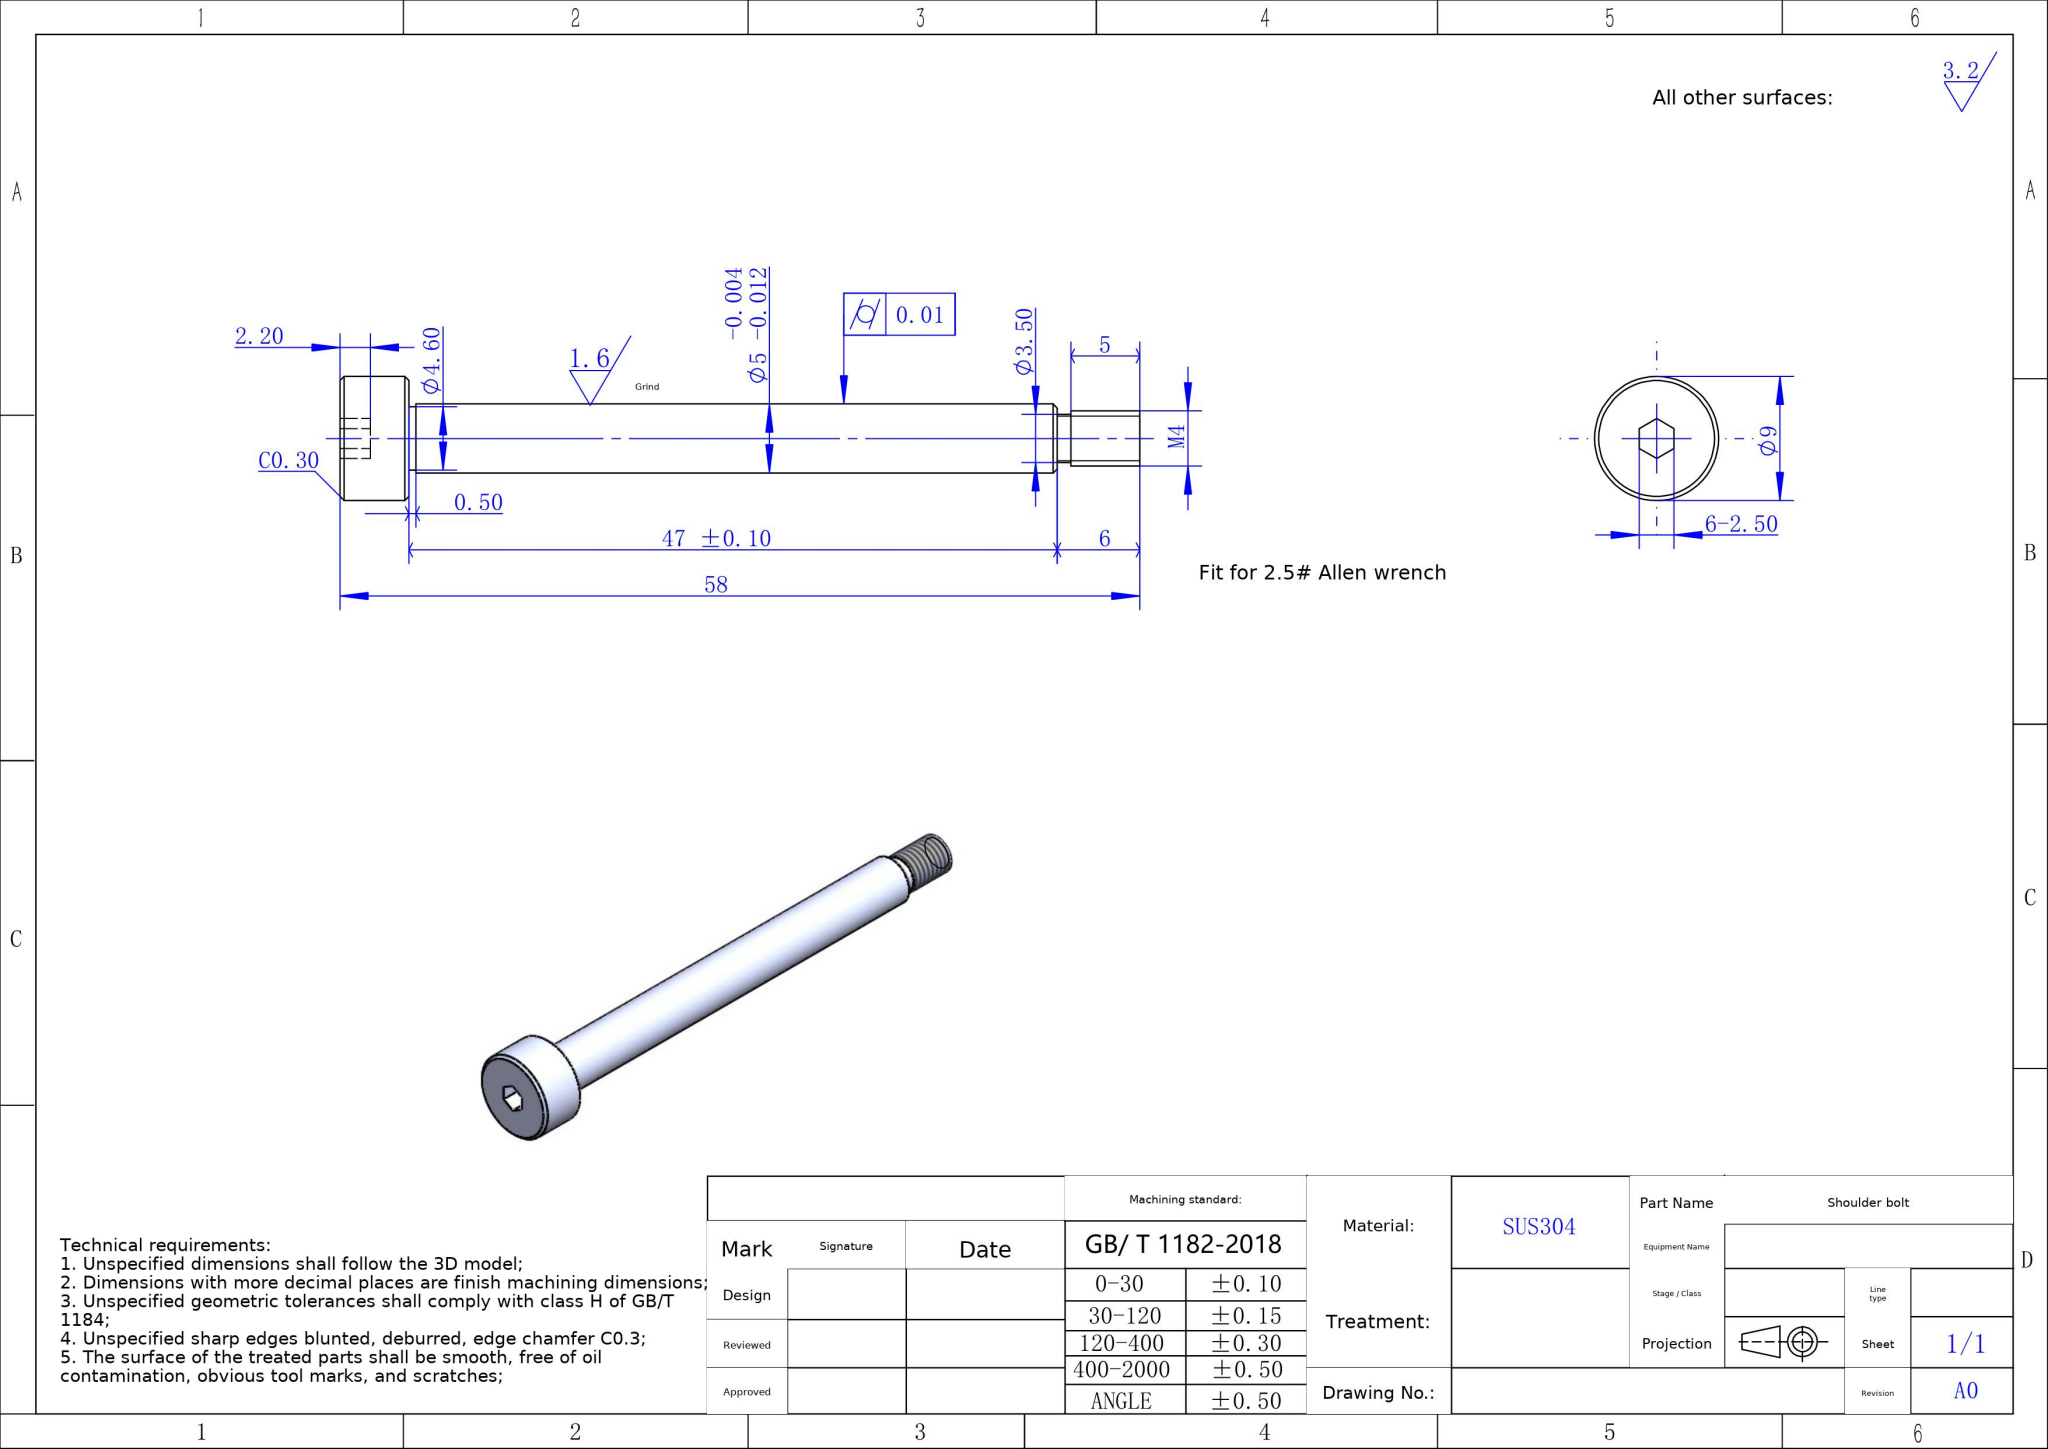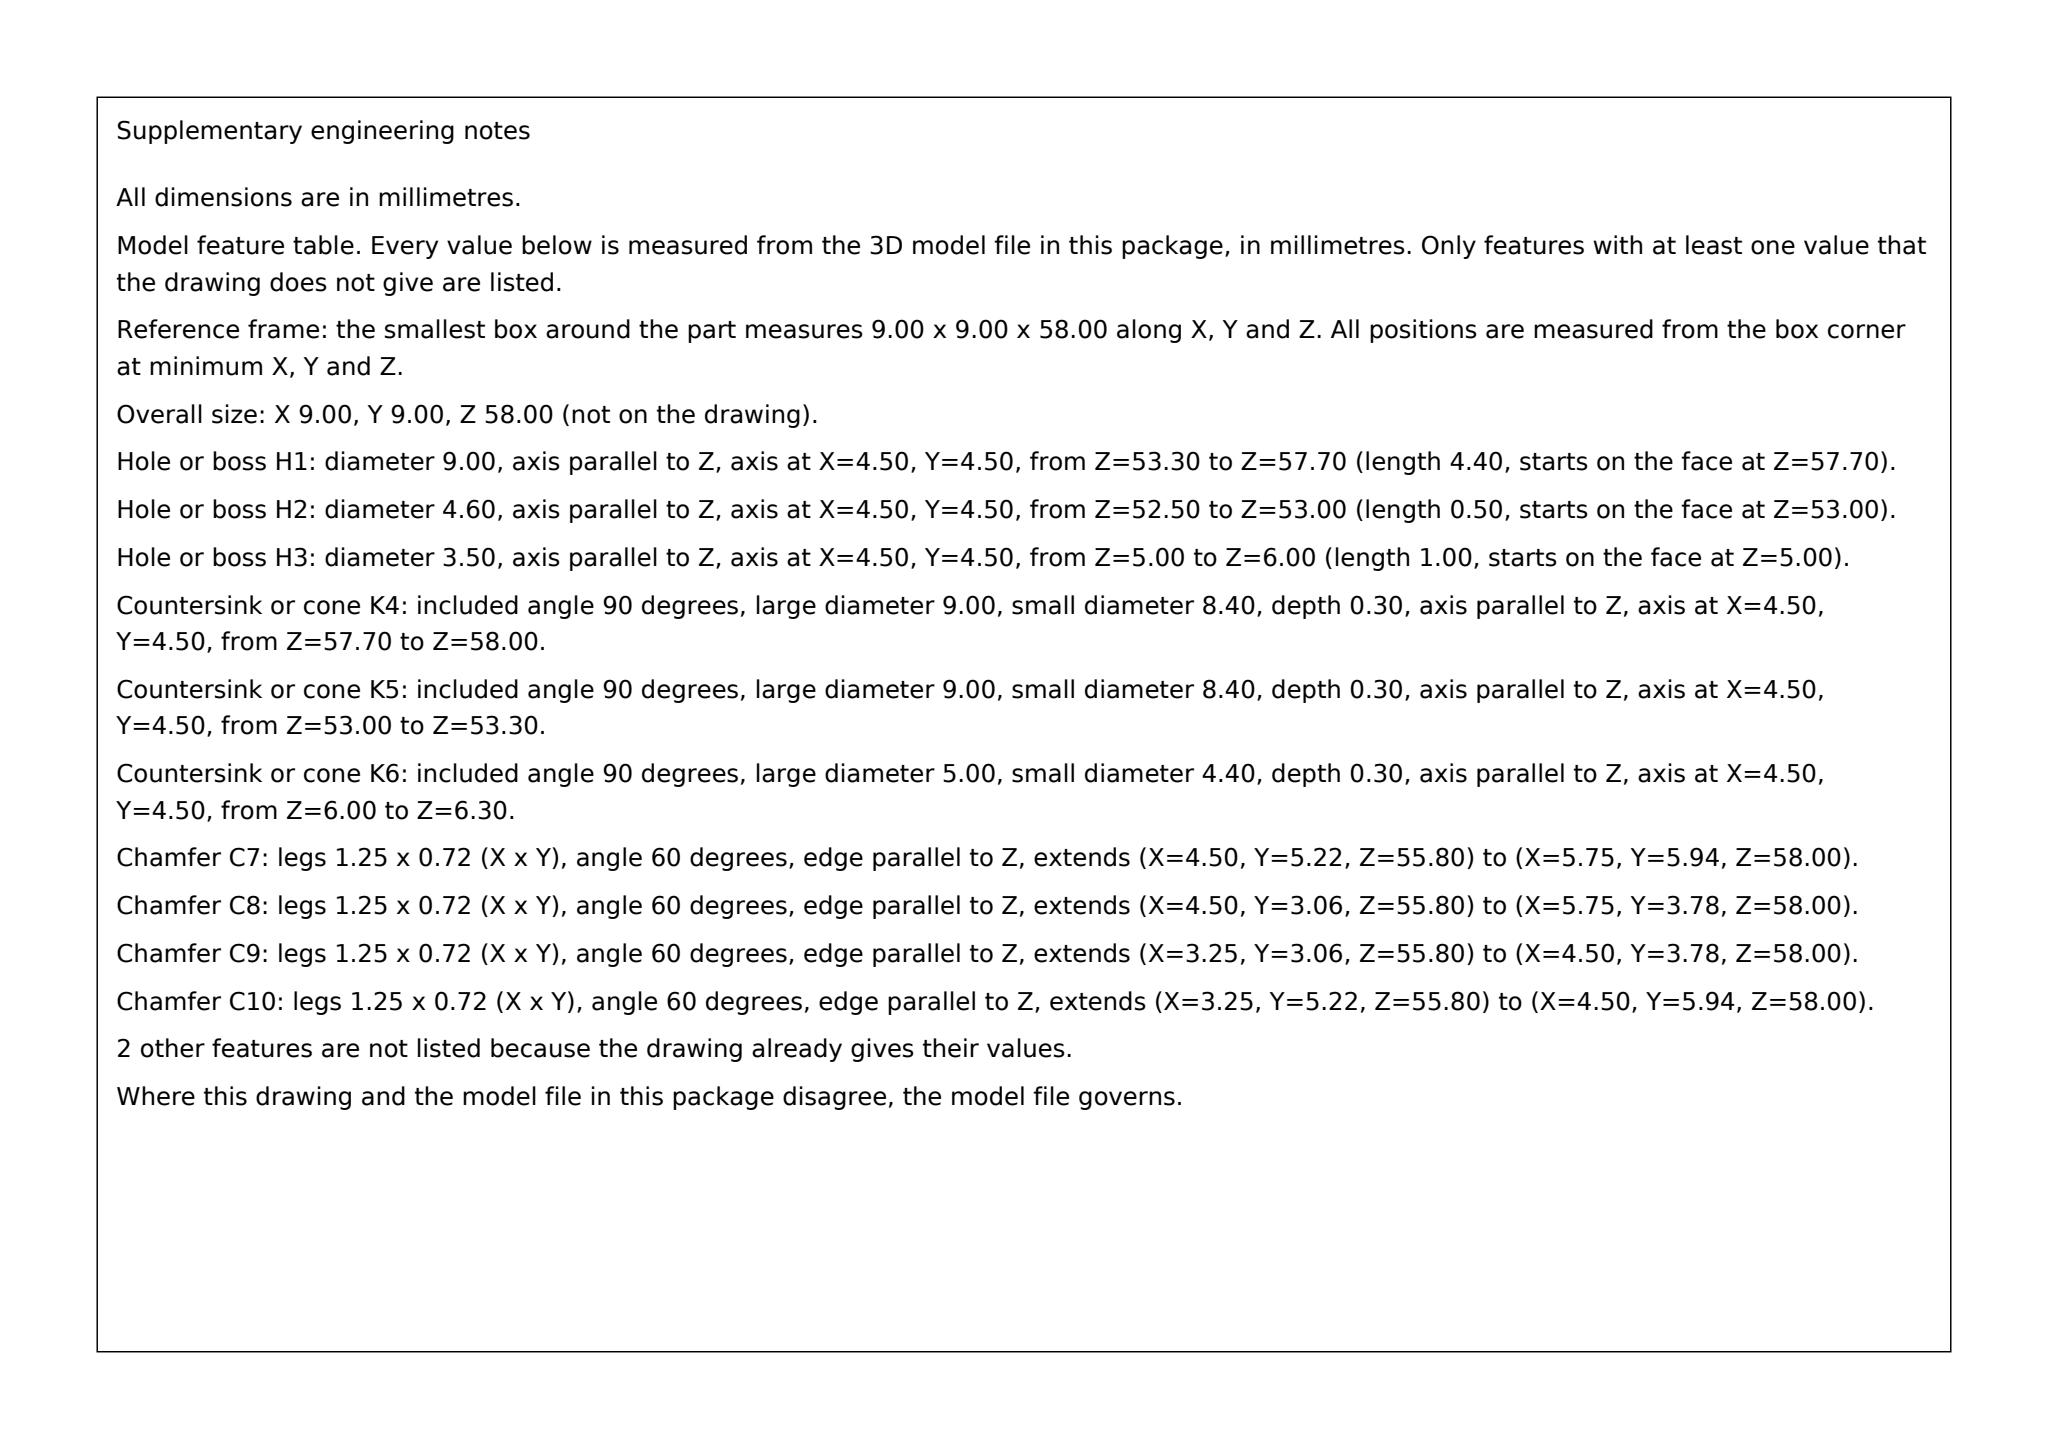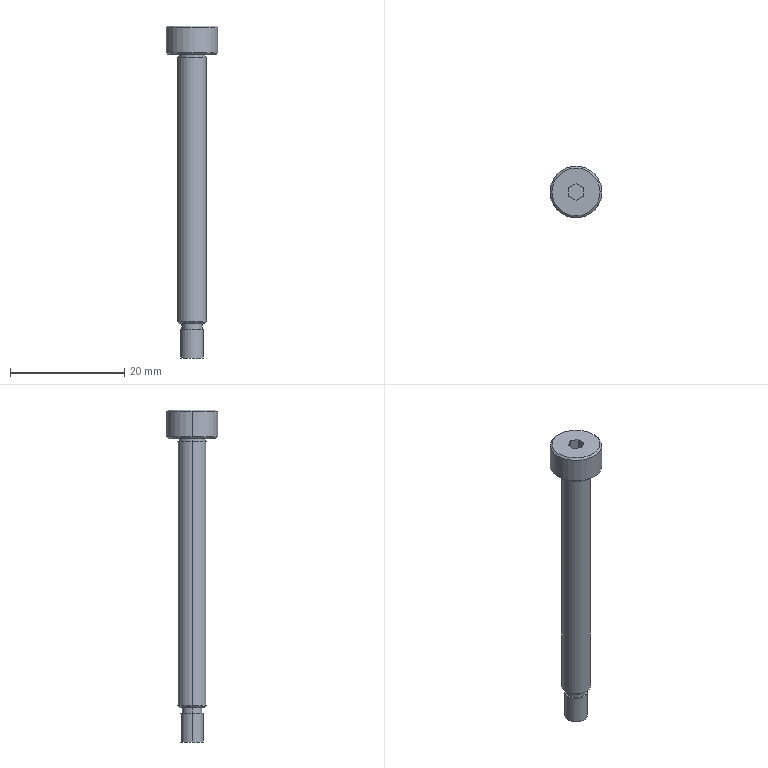Part | SolidWorks | mm | material SUS304 | 1 solid | 29 faces | box 9 x 9 x 58 mm | volume 1297 mm3 | plane 13 | cylinder 10 | cone 6 | commonest cylinder face diameters 4 x2 3.5 x2 5 x2 4.6 x2 9 x2
build123d program:
from build123d import *

# Parameters (mm, degrees)
SKETCH1_R           = 4.5
BOSS_EXTRUDE1_DEPTH = 5
SKETCH2_R           = 2.5
BOSS_EXTRUDE2_DEPTH = 47
SKETCH3_R           = 2
BOSS_EXTRUDE3_DEPTH = 6
SKETCH4_W           = 0.486
SKETCH4_H           = 1
SKETCH4_W_2         = 0.3002
SKETCH4_H_2         = 0.5
CUT_EXTRUDE1_DEPTH  = 2.2
CHAMFER1_SIZE       = 0.3


with BuildPart() as part:
    # Sketch1 → Boss-Extrude1 (new body)
    with BuildSketch(Plane.XY):
        Circle(SKETCH1_R)
    extrude(amount=BOSS_EXTRUDE1_DEPTH)

    # Sketch2 → Boss-Extrude2 (add)
    with BuildSketch(Plane(origin=(0, 0, 0), x_dir=(-1, 0, 0), z_dir=(0, 0, -1))):
        Circle(SKETCH2_R)
    extrude(amount=BOSS_EXTRUDE2_DEPTH)

    # Sketch3 → Boss-Extrude3 (add)
    with BuildSketch(Plane(origin=(0, 0, -47), x_dir=(-1, 0, 0), z_dir=(0, 0, -1))):
        Circle(SKETCH3_R)
    extrude(amount=BOSS_EXTRUDE3_DEPTH)

    # Sketch4 → Cut-Revolve1 (revolve, cut)
    with BuildSketch(Plane(origin=(0, 0, 0), x_dir=(1, 0, 0), z_dir=(0, 1, 0))):
        with Locations((1.993, 47.5)):
            Rectangle(SKETCH4_W, SKETCH4_H)
        with Locations((2.45, 0.25)):
            Rectangle(SKETCH4_W_2, SKETCH4_H_2)
    revolve(axis=Axis((0, 0, -53), (0, 0, -1)), mode=Mode.SUBTRACT)

    # Sketch5 → Cut-Extrude1 (cut)
    with BuildSketch(Plane.XY.offset(5)):
        Polygon((0, 1.443), (-1.25, 0.7217), (-1.25, -0.7217), (0, -1.443), (1.25, -0.7217), (1.25, 0.7217), align=None)
    extrude(amount=-CUT_EXTRUDE1_DEPTH, mode=Mode.SUBTRACT)

    # Chamfer1
    chamfer1_edges = [part.edges().sort_by_distance(p)[0] for p in [
        (-4.5, 0, 0),
        (-4.5, 0, 5),
        (2.5, 0, -47),
    ]]
    chamfer(chamfer1_edges, length=CHAMFER1_SIZE)


solid = part.part
STEP:
#1=CARTESIAN_POINT('',(4.2,0.,5.));
#2=VERTEX_POINT('',#1);
#3=CARTESIAN_POINT('',(-4.2,0.,5.));
#4=VERTEX_POINT('',#3);
#5=CARTESIAN_POINT('',(0.,0.,5.));
#6=DIRECTION('',(0.,0.,1.));
#7=DIRECTION('',(1.,0.,0.));
#8=AXIS2_PLACEMENT_3D('',#5,#6,#7);
#9=CIRCLE('',#8,4.2);
#10=EDGE_CURVE('',#2,#4,#9,.T.);
#11=ORIENTED_EDGE('',*,*,#10,.F.);
#12=CARTESIAN_POINT('',(4.5,0.,4.7));
#13=VERTEX_POINT('',#12);
#14=CARTESIAN_POINT('',(4.2,0.,5.));
#15=DIRECTION('',(0.7071,0.,-0.7071));
#16=VECTOR('',#15,1000.);
#17=LINE('',#14,#16);
#18=EDGE_CURVE('',#2,#13,#17,.T.);
#19=ORIENTED_EDGE('',*,*,#18,.T.);
#20=CARTESIAN_POINT('',(-4.5,0.,4.7));
#21=VERTEX_POINT('',#20);
#22=CARTESIAN_POINT('',(0.,0.,4.7));
#23=DIRECTION('',(0.,0.,-1.));
#24=DIRECTION('',(1.,0.,0.));
#25=AXIS2_PLACEMENT_3D('',#22,#23,#24);
#26=CIRCLE('',#25,4.5);
#27=EDGE_CURVE('',#21,#13,#26,.T.);
#28=ORIENTED_EDGE('',*,*,#27,.F.);
#29=CARTESIAN_POINT('',(-4.2,0.,5.));
#30=DIRECTION('',(-0.7071,0.,-0.7071));
#31=VECTOR('',#30,1000.);
#32=LINE('',#29,#31);
#33=EDGE_CURVE('',#4,#21,#32,.T.);
#34=ORIENTED_EDGE('',*,*,#33,.F.);
#35=EDGE_LOOP('',(#11,#19,#28,#34));
#36=FACE_OUTER_BOUND('',#35,.T.);
#37=CARTESIAN_POINT('',(0.,0.,5.));
#38=DIRECTION('',(0.,0.,-1.));
#39=DIRECTION('',(-1.,0.,0.));
#40=AXIS2_PLACEMENT_3D('',#37,#38,#39);
#41=CONICAL_SURFACE('',#40,4.2,0.7854);
#42=ADVANCED_FACE('',(#36),#41,.T.);
#43=CARTESIAN_POINT('',(-4.2,0.,0.));
#44=VERTEX_POINT('',#43);
#45=CARTESIAN_POINT('',(4.2,0.,0.));
#46=VERTEX_POINT('',#45);
#47=CARTESIAN_POINT('',(0.,0.,0.));
#48=DIRECTION('',(0.,0.,-1.));
#49=DIRECTION('',(1.,0.,0.));
#50=AXIS2_PLACEMENT_3D('',#47,#48,#49);
#51=CIRCLE('',#50,4.2);
#52=EDGE_CURVE('',#44,#46,#51,.T.);
#53=ORIENTED_EDGE('',*,*,#52,.F.);
#54=CARTESIAN_POINT('',(-4.5,0.,0.3));
#55=VERTEX_POINT('',#54);
#56=CARTESIAN_POINT('',(-4.5,0.,0.3));
#57=DIRECTION('',(-0.7071,0.,0.7071));
#58=VECTOR('',#57,1000.);
#59=LINE('',#56,#58);
#60=EDGE_CURVE('',#44,#55,#59,.T.);
#61=ORIENTED_EDGE('',*,*,#60,.T.);
#62=CARTESIAN_POINT('',(4.5,0.,0.3));
#63=VERTEX_POINT('',#62);
#64=CARTESIAN_POINT('',(0.,0.,0.3));
#65=DIRECTION('',(0.,0.,1.));
#66=DIRECTION('',(1.,0.,0.));
#67=AXIS2_PLACEMENT_3D('',#64,#65,#66);
#68=CIRCLE('',#67,4.5);
#69=EDGE_CURVE('',#63,#55,#68,.T.);
#70=ORIENTED_EDGE('',*,*,#69,.F.);
#71=CARTESIAN_POINT('',(4.5,0.,0.3));
#72=DIRECTION('',(0.7071,0.,0.7071));
#73=VECTOR('',#72,1000.);
#74=LINE('',#71,#73);
#75=EDGE_CURVE('',#46,#63,#74,.T.);
#76=ORIENTED_EDGE('',*,*,#75,.F.);
#77=EDGE_LOOP('',(#53,#61,#70,#76));
#78=FACE_OUTER_BOUND('',#77,.T.);
#79=CARTESIAN_POINT('',(0.,0.,0.3));
#80=DIRECTION('',(0.,0.,1.));
#81=DIRECTION('',(1.,0.,0.));
#82=AXIS2_PLACEMENT_3D('',#79,#80,#81);
#83=CONICAL_SURFACE('',#82,4.5,0.7854);
#84=ADVANCED_FACE('',(#78),#83,.T.);
#85=CARTESIAN_POINT('',(-2.2,0.,-47.));
#86=VERTEX_POINT('',#85);
#87=CARTESIAN_POINT('',(2.2,0.,-47.));
#88=VERTEX_POINT('',#87);
#89=CARTESIAN_POINT('',(0.,0.,-47.));
#90=DIRECTION('',(0.,0.,-1.));
#91=DIRECTION('',(-1.,0.,0.));
#92=AXIS2_PLACEMENT_3D('',#89,#90,#91);
#93=CIRCLE('',#92,2.2);
#94=EDGE_CURVE('',#86,#88,#93,.T.);
#95=ORIENTED_EDGE('',*,*,#94,.F.);
#96=CARTESIAN_POINT('',(-2.5,0.,-46.7));
#97=VERTEX_POINT('',#96);
#98=CARTESIAN_POINT('',(-2.2,0.,-47.));
#99=DIRECTION('',(-0.7071,0.,0.7071));
#100=VECTOR('',#99,1000.);
#101=LINE('',#98,#100);
#102=EDGE_CURVE('',#86,#97,#101,.T.);
#103=ORIENTED_EDGE('',*,*,#102,.T.);
#104=CARTESIAN_POINT('',(2.5,0.,-46.7));
#105=VERTEX_POINT('',#104);
#106=CARTESIAN_POINT('',(0.,0.,-46.7));
#107=DIRECTION('',(0.,0.,1.));
#108=DIRECTION('',(-1.,0.,0.));
#109=AXIS2_PLACEMENT_3D('',#106,#107,#108);
#110=CIRCLE('',#109,2.5);
#111=EDGE_CURVE('',#105,#97,#110,.T.);
#112=ORIENTED_EDGE('',*,*,#111,.F.);
#113=CARTESIAN_POINT('',(2.2,0.,-47.));
#114=DIRECTION('',(0.7071,0.,0.7071));
#115=VECTOR('',#114,1000.);
#116=LINE('',#113,#115);
#117=EDGE_CURVE('',#88,#105,#116,.T.);
#118=ORIENTED_EDGE('',*,*,#117,.F.);
#119=EDGE_LOOP('',(#95,#103,#112,#118));
#120=FACE_OUTER_BOUND('',#119,.T.);
#121=CARTESIAN_POINT('',(0.,0.,-47.));
#122=DIRECTION('',(0.,0.,1.));
#123=DIRECTION('',(1.,0.,0.));
#124=AXIS2_PLACEMENT_3D('',#121,#122,#123);
#125=CONICAL_SURFACE('',#124,2.2,0.7854);
#126=ADVANCED_FACE('',(#120),#125,.T.);
#127=CARTESIAN_POINT('',(-2.,0.,-53.));
#128=VERTEX_POINT('',#127);
#129=CARTESIAN_POINT('',(2.,0.,-53.));
#130=VERTEX_POINT('',#129);
#131=CARTESIAN_POINT('',(0.,0.,-53.));
#132=DIRECTION('',(0.,0.,-1.));
#133=DIRECTION('',(-1.,0.,0.));
#134=AXIS2_PLACEMENT_3D('',#131,#132,#133);
#135=CIRCLE('',#134,2.);
#136=EDGE_CURVE('',#128,#130,#135,.T.);
#137=ORIENTED_EDGE('',*,*,#136,.F.);
#138=CARTESIAN_POINT('',(-2.,0.,-48.));
#139=VERTEX_POINT('',#138);
#140=CARTESIAN_POINT('',(-2.,0.,-53.));
#141=DIRECTION('',(0.,0.,1.));
#142=VECTOR('',#141,1000.);
#143=LINE('',#140,#142);
#144=EDGE_CURVE('',#128,#139,#143,.T.);
#145=ORIENTED_EDGE('',*,*,#144,.T.);
#146=CARTESIAN_POINT('',(2.,0.,-48.));
#147=VERTEX_POINT('',#146);
#148=CARTESIAN_POINT('',(0.,0.,-48.));
#149=DIRECTION('',(0.,0.,-1.));
#150=DIRECTION('',(-1.,0.,0.));
#151=AXIS2_PLACEMENT_3D('',#148,#149,#150);
#152=CIRCLE('',#151,2.);
#153=EDGE_CURVE('',#139,#147,#152,.T.);
#154=ORIENTED_EDGE('',*,*,#153,.T.);
#155=CARTESIAN_POINT('',(2.,0.,-53.));
#156=DIRECTION('',(0.,0.,1.));
#157=VECTOR('',#156,1000.);
#158=LINE('',#155,#157);
#159=EDGE_CURVE('',#130,#147,#158,.T.);
#160=ORIENTED_EDGE('',*,*,#159,.F.);
#161=EDGE_LOOP('',(#137,#145,#154,#160));
#162=FACE_OUTER_BOUND('',#161,.T.);
#163=CARTESIAN_POINT('',(0.,0.,-53.));
#164=DIRECTION('',(0.,0.,1.));
#165=DIRECTION('',(1.,0.,0.));
#166=AXIS2_PLACEMENT_3D('',#163,#164,#165);
#167=CYLINDRICAL_SURFACE('',#166,2.);
#168=ADVANCED_FACE('',(#162),#167,.T.);
#169=CARTESIAN_POINT('',(1.75,0.,-48.));
#170=VERTEX_POINT('',#169);
#171=CARTESIAN_POINT('',(-1.75,0.,-48.));
#172=VERTEX_POINT('',#171);
#173=CARTESIAN_POINT('',(0.,0.,-48.));
#174=DIRECTION('',(0.,0.,1.));
#175=DIRECTION('',(1.,0.,0.));
#176=AXIS2_PLACEMENT_3D('',#173,#174,#175);
#177=CIRCLE('',#176,1.75);
#178=EDGE_CURVE('',#170,#172,#177,.T.);
#179=ORIENTED_EDGE('',*,*,#178,.T.);
#180=CARTESIAN_POINT('',(-1.75,0.,-47.));
#181=VERTEX_POINT('',#180);
#182=CARTESIAN_POINT('',(-1.75,0.,-53.));
#183=DIRECTION('',(0.,0.,1.));
#184=VECTOR('',#183,1000.);
#185=LINE('',#182,#184);
#186=EDGE_CURVE('',#172,#181,#185,.T.);
#187=ORIENTED_EDGE('',*,*,#186,.T.);
#188=CARTESIAN_POINT('',(1.75,0.,-47.));
#189=VERTEX_POINT('',#188);
#190=CARTESIAN_POINT('',(0.,0.,-47.));
#191=DIRECTION('',(0.,0.,1.));
#192=DIRECTION('',(1.,0.,0.));
#193=AXIS2_PLACEMENT_3D('',#190,#191,#192);
#194=CIRCLE('',#193,1.75);
#195=EDGE_CURVE('',#189,#181,#194,.T.);
#196=ORIENTED_EDGE('',*,*,#195,.F.);
#197=CARTESIAN_POINT('',(1.75,0.,-53.));
#198=DIRECTION('',(0.,0.,1.));
#199=VECTOR('',#198,1000.);
#200=LINE('',#197,#199);
#201=EDGE_CURVE('',#170,#189,#200,.T.);
#202=ORIENTED_EDGE('',*,*,#201,.F.);
#203=EDGE_LOOP('',(#179,#187,#196,#202));
#204=FACE_OUTER_BOUND('',#203,.T.);
#205=CARTESIAN_POINT('',(0.,0.,-53.));
#206=DIRECTION('',(0.,0.,1.));
#207=DIRECTION('',(1.,0.,0.));
#208=AXIS2_PLACEMENT_3D('',#205,#206,#207);
#209=CYLINDRICAL_SURFACE('',#208,1.75);
#210=ADVANCED_FACE('',(#204),#209,.T.);
#211=ORIENTED_EDGE('',*,*,#111,.T.);
#212=CARTESIAN_POINT('',(-2.5,0.,-0.5));
#213=VERTEX_POINT('',#212);
#214=CARTESIAN_POINT('',(-2.5,0.,-47.));
#215=DIRECTION('',(0.,0.,1.));
#216=VECTOR('',#215,1000.);
#217=LINE('',#214,#216);
#218=EDGE_CURVE('',#97,#213,#217,.T.);
#219=ORIENTED_EDGE('',*,*,#218,.T.);
#220=CARTESIAN_POINT('',(2.5,0.,-0.5));
#221=VERTEX_POINT('',#220);
#222=CARTESIAN_POINT('',(0.,0.,-0.5));
#223=DIRECTION('',(0.,0.,-1.));
#224=DIRECTION('',(-1.,0.,0.));
#225=AXIS2_PLACEMENT_3D('',#222,#223,#224);
#226=CIRCLE('',#225,2.5);
#227=EDGE_CURVE('',#213,#221,#226,.T.);
#228=ORIENTED_EDGE('',*,*,#227,.T.);
#229=CARTESIAN_POINT('',(2.5,0.,-47.));
#230=DIRECTION('',(0.,0.,1.));
#231=VECTOR('',#230,1000.);
#232=LINE('',#229,#231);
#233=EDGE_CURVE('',#105,#221,#232,.T.);
#234=ORIENTED_EDGE('',*,*,#233,.F.);
#235=EDGE_LOOP('',(#211,#219,#228,#234));
#236=FACE_OUTER_BOUND('',#235,.T.);
#237=CARTESIAN_POINT('',(0.,0.,-47.));
#238=DIRECTION('',(0.,0.,1.));
#239=DIRECTION('',(1.,0.,0.));
#240=AXIS2_PLACEMENT_3D('',#237,#238,#239);
#241=CYLINDRICAL_SURFACE('',#240,2.5);
#242=ADVANCED_FACE('',(#236),#241,.T.);
#243=CARTESIAN_POINT('',(2.3,0.,-0.5));
#244=VERTEX_POINT('',#243);
#245=CARTESIAN_POINT('',(-2.3,0.,-0.5));
#246=VERTEX_POINT('',#245);
#247=CARTESIAN_POINT('',(0.,0.,-0.5));
#248=DIRECTION('',(0.,0.,1.));
#249=DIRECTION('',(1.,0.,0.));
#250=AXIS2_PLACEMENT_3D('',#247,#248,#249);
#251=CIRCLE('',#250,2.3);
#252=EDGE_CURVE('',#244,#246,#251,.T.);
#253=ORIENTED_EDGE('',*,*,#252,.T.);
#254=CARTESIAN_POINT('',(-2.3,0.,0.));
#255=VERTEX_POINT('',#254);
#256=CARTESIAN_POINT('',(-2.3,0.,-53.));
#257=DIRECTION('',(0.,0.,1.));
#258=VECTOR('',#257,1000.);
#259=LINE('',#256,#258);
#260=EDGE_CURVE('',#246,#255,#259,.T.);
#261=ORIENTED_EDGE('',*,*,#260,.T.);
#262=CARTESIAN_POINT('',(2.3,0.,0.));
#263=VERTEX_POINT('',#262);
#264=CARTESIAN_POINT('',(0.,0.,0.));
#265=DIRECTION('',(0.,0.,1.));
#266=DIRECTION('',(1.,0.,0.));
#267=AXIS2_PLACEMENT_3D('',#264,#265,#266);
#268=CIRCLE('',#267,2.3);
#269=EDGE_CURVE('',#263,#255,#268,.T.);
#270=ORIENTED_EDGE('',*,*,#269,.F.);
#271=CARTESIAN_POINT('',(2.3,0.,-53.));
#272=DIRECTION('',(0.,0.,1.));
#273=VECTOR('',#272,1000.);
#274=LINE('',#271,#273);
#275=EDGE_CURVE('',#244,#263,#274,.T.);
#276=ORIENTED_EDGE('',*,*,#275,.F.);
#277=EDGE_LOOP('',(#253,#261,#270,#276));
#278=FACE_OUTER_BOUND('',#277,.T.);
#279=CARTESIAN_POINT('',(0.,0.,-53.));
#280=DIRECTION('',(0.,0.,1.));
#281=DIRECTION('',(1.,0.,0.));
#282=AXIS2_PLACEMENT_3D('',#279,#280,#281);
#283=CYLINDRICAL_SURFACE('',#282,2.3);
#284=ADVANCED_FACE('',(#278),#283,.T.);
#285=ORIENTED_EDGE('',*,*,#27,.T.);
#286=CARTESIAN_POINT('',(4.5,0.,5.));
#287=DIRECTION('',(0.,0.,-1.));
#288=VECTOR('',#287,1000.);
#289=LINE('',#286,#288);
#290=EDGE_CURVE('',#13,#63,#289,.T.);
#291=ORIENTED_EDGE('',*,*,#290,.T.);
#292=ORIENTED_EDGE('',*,*,#69,.T.);
#293=CARTESIAN_POINT('',(-4.5,0.,5.));
#294=DIRECTION('',(0.,0.,-1.));
#295=VECTOR('',#294,1000.);
#296=LINE('',#293,#295);
#297=EDGE_CURVE('',#21,#55,#296,.T.);
#298=ORIENTED_EDGE('',*,*,#297,.F.);
#299=EDGE_LOOP('',(#285,#291,#292,#298));
#300=FACE_OUTER_BOUND('',#299,.T.);
#301=CARTESIAN_POINT('',(0.,0.,5.));
#302=DIRECTION('',(0.,0.,-1.));
#303=DIRECTION('',(-1.,0.,0.));
#304=AXIS2_PLACEMENT_3D('',#301,#302,#303);
#305=CYLINDRICAL_SURFACE('',#304,4.5);
#306=ADVANCED_FACE('',(#300),#305,.T.);
#307=ORIENTED_EDGE('',*,*,#290,.F.);
#308=CARTESIAN_POINT('',(0.,0.,4.7));
#309=DIRECTION('',(0.,0.,-1.));
#310=DIRECTION('',(1.,0.,0.));
#311=AXIS2_PLACEMENT_3D('',#308,#309,#310);
#312=CIRCLE('',#311,4.5);
#313=EDGE_CURVE('',#13,#21,#312,.T.);
#314=ORIENTED_EDGE('',*,*,#313,.T.);
#315=ORIENTED_EDGE('',*,*,#297,.T.);
#316=CARTESIAN_POINT('',(0.,0.,0.3));
#317=DIRECTION('',(0.,0.,1.));
#318=DIRECTION('',(1.,0.,0.));
#319=AXIS2_PLACEMENT_3D('',#316,#317,#318);
#320=CIRCLE('',#319,4.5);
#321=EDGE_CURVE('',#55,#63,#320,.T.);
#322=ORIENTED_EDGE('',*,*,#321,.T.);
#323=EDGE_LOOP('',(#307,#314,#315,#322));
#324=FACE_OUTER_BOUND('',#323,.T.);
#325=CARTESIAN_POINT('',(0.,0.,5.));
#326=DIRECTION('',(0.,0.,-1.));
#327=DIRECTION('',(-1.,0.,0.));
#328=AXIS2_PLACEMENT_3D('',#325,#326,#327);
#329=CYLINDRICAL_SURFACE('',#328,4.5);
#330=ADVANCED_FACE('',(#324),#329,.T.);
#331=CARTESIAN_POINT('',(0.,0.,5.));
#332=DIRECTION('',(0.,0.,1.));
#333=DIRECTION('',(1.,0.,0.));
#334=AXIS2_PLACEMENT_3D('',#331,#332,#333);
#335=CIRCLE('',#334,4.2);
#336=EDGE_CURVE('',#4,#2,#335,.T.);
#337=ORIENTED_EDGE('',*,*,#336,.T.);
#338=ORIENTED_EDGE('',*,*,#10,.T.);
#339=EDGE_LOOP('',(#337,#338));
#340=FACE_OUTER_BOUND('',#339,.T.);
#341=CARTESIAN_POINT('',(1.25,0.7217,5.));
#342=VERTEX_POINT('',#341);
#343=CARTESIAN_POINT('',(0.,1.443,5.));
#344=VERTEX_POINT('',#343);
#345=CARTESIAN_POINT('',(1.25,0.7217,5.));
#346=DIRECTION('',(-0.866,0.5,0.));
#347=VECTOR('',#346,1000.);
#348=LINE('',#345,#347);
#349=EDGE_CURVE('',#342,#344,#348,.T.);
#350=ORIENTED_EDGE('',*,*,#349,.F.);
#351=CARTESIAN_POINT('',(1.25,-0.7217,5.));
#352=VERTEX_POINT('',#351);
#353=CARTESIAN_POINT('',(1.25,-0.7217,5.));
#354=DIRECTION('',(0.,1.,0.));
#355=VECTOR('',#354,1000.);
#356=LINE('',#353,#355);
#357=EDGE_CURVE('',#352,#342,#356,.T.);
#358=ORIENTED_EDGE('',*,*,#357,.F.);
#359=CARTESIAN_POINT('',(0.,-1.443,5.));
#360=VERTEX_POINT('',#359);
#361=CARTESIAN_POINT('',(0.,-1.443,5.));
#362=DIRECTION('',(0.866,0.5,0.));
#363=VECTOR('',#362,1000.);
#364=LINE('',#361,#363);
#365=EDGE_CURVE('',#360,#352,#364,.T.);
#366=ORIENTED_EDGE('',*,*,#365,.F.);
#367=CARTESIAN_POINT('',(-1.25,-0.7217,5.));
#368=VERTEX_POINT('',#367);
#369=CARTESIAN_POINT('',(-1.25,-0.7217,5.));
#370=DIRECTION('',(0.866,-0.5,0.));
#371=VECTOR('',#370,1000.);
#372=LINE('',#369,#371);
#373=EDGE_CURVE('',#368,#360,#372,.T.);
#374=ORIENTED_EDGE('',*,*,#373,.F.);
#375=CARTESIAN_POINT('',(-1.25,0.7217,5.));
#376=VERTEX_POINT('',#375);
#377=CARTESIAN_POINT('',(-1.25,0.7217,5.));
#378=DIRECTION('',(0.,-1.,0.));
#379=VECTOR('',#378,1000.);
#380=LINE('',#377,#379);
#381=EDGE_CURVE('',#376,#368,#380,.T.);
#382=ORIENTED_EDGE('',*,*,#381,.F.);
#383=CARTESIAN_POINT('',(0.,1.443,5.));
#384=DIRECTION('',(-0.866,-0.5,0.));
#385=VECTOR('',#384,1000.);
#386=LINE('',#383,#385);
#387=EDGE_CURVE('',#344,#376,#386,.T.);
#388=ORIENTED_EDGE('',*,*,#387,.F.);
#389=EDGE_LOOP('',(#350,#358,#366,#374,#382,#388));
#390=FACE_BOUND('',#389,.T.);
#391=CARTESIAN_POINT('',(0.,0.,5.));
#392=DIRECTION('',(0.,0.,1.));
#393=DIRECTION('',(1.,0.,0.));
#394=AXIS2_PLACEMENT_3D('',#391,#392,#393);
#395=PLANE('',#394);
#396=ADVANCED_FACE('',(#340,#390),#395,.T.);
#397=CARTESIAN_POINT('',(0.,0.,0.));
#398=DIRECTION('',(0.,0.,-1.));
#399=DIRECTION('',(1.,0.,0.));
#400=AXIS2_PLACEMENT_3D('',#397,#398,#399);
#401=CIRCLE('',#400,4.2);
#402=EDGE_CURVE('',#46,#44,#401,.T.);
#403=ORIENTED_EDGE('',*,*,#402,.T.);
#404=ORIENTED_EDGE('',*,*,#52,.T.);
#405=EDGE_LOOP('',(#403,#404));
#406=FACE_OUTER_BOUND('',#405,.T.);
#407=ORIENTED_EDGE('',*,*,#269,.T.);
#408=CARTESIAN_POINT('',(0.,0.,0.));
#409=DIRECTION('',(0.,0.,1.));
#410=DIRECTION('',(1.,0.,0.));
#411=AXIS2_PLACEMENT_3D('',#408,#409,#410);
#412=CIRCLE('',#411,2.3);
#413=EDGE_CURVE('',#255,#263,#412,.T.);
#414=ORIENTED_EDGE('',*,*,#413,.T.);
#415=EDGE_LOOP('',(#407,#414));
#416=FACE_BOUND('',#415,.T.);
#417=CARTESIAN_POINT('',(0.,0.,0.));
#418=DIRECTION('',(0.,0.,1.));
#419=DIRECTION('',(1.,0.,0.));
#420=AXIS2_PLACEMENT_3D('',#417,#418,#419);
#421=PLANE('',#420);
#422=ADVANCED_FACE('',(#406,#416),#421,.F.);
#423=ORIENTED_EDGE('',*,*,#252,.F.);
#424=CARTESIAN_POINT('',(0.,0.,-0.5));
#425=DIRECTION('',(0.,0.,1.));
#426=DIRECTION('',(1.,0.,0.));
#427=AXIS2_PLACEMENT_3D('',#424,#425,#426);
#428=CIRCLE('',#427,2.3);
#429=EDGE_CURVE('',#246,#244,#428,.T.);
#430=ORIENTED_EDGE('',*,*,#429,.F.);
#431=EDGE_LOOP('',(#423,#430));
#432=FACE_BOUND('',#431,.T.);
#433=CARTESIAN_POINT('',(0.,0.,-0.5));
#434=DIRECTION('',(0.,0.,-1.));
#435=DIRECTION('',(-1.,0.,0.));
#436=AXIS2_PLACEMENT_3D('',#433,#434,#435);
#437=CIRCLE('',#436,2.5);
#438=EDGE_CURVE('',#221,#213,#437,.T.);
#439=ORIENTED_EDGE('',*,*,#438,.F.);
#440=ORIENTED_EDGE('',*,*,#227,.F.);
#441=EDGE_LOOP('',(#439,#440));
#442=FACE_OUTER_BOUND('',#441,.T.);
#443=CARTESIAN_POINT('',(2.6,0.,-0.5));
#444=DIRECTION('',(0.,0.,-1.));
#445=DIRECTION('',(-1.,0.,0.));
#446=AXIS2_PLACEMENT_3D('',#443,#444,#445);
#447=PLANE('',#446);
#448=ADVANCED_FACE('',(#432,#442),#447,.F.);
#449=ORIENTED_EDGE('',*,*,#260,.F.);
#450=ORIENTED_EDGE('',*,*,#429,.T.);
#451=ORIENTED_EDGE('',*,*,#275,.T.);
#452=ORIENTED_EDGE('',*,*,#413,.F.);
#453=EDGE_LOOP('',(#449,#450,#451,#452));
#454=FACE_OUTER_BOUND('',#453,.T.);
#455=CARTESIAN_POINT('',(0.,0.,-53.));
#456=DIRECTION('',(0.,0.,1.));
#457=DIRECTION('',(1.,0.,0.));
#458=AXIS2_PLACEMENT_3D('',#455,#456,#457);
#459=CYLINDRICAL_SURFACE('',#458,2.3);
#460=ADVANCED_FACE('',(#454),#459,.T.);
#461=ORIENTED_EDGE('',*,*,#218,.F.);
#462=CARTESIAN_POINT('',(0.,0.,-46.7));
#463=DIRECTION('',(0.,0.,1.));
#464=DIRECTION('',(-1.,0.,0.));
#465=AXIS2_PLACEMENT_3D('',#462,#463,#464);
#466=CIRCLE('',#465,2.5);
#467=EDGE_CURVE('',#97,#105,#466,.T.);
#468=ORIENTED_EDGE('',*,*,#467,.T.);
#469=ORIENTED_EDGE('',*,*,#233,.T.);
#470=ORIENTED_EDGE('',*,*,#438,.T.);
#471=EDGE_LOOP('',(#461,#468,#469,#470));
#472=FACE_OUTER_BOUND('',#471,.T.);
#473=CARTESIAN_POINT('',(0.,0.,-47.));
#474=DIRECTION('',(0.,0.,1.));
#475=DIRECTION('',(1.,0.,0.));
#476=AXIS2_PLACEMENT_3D('',#473,#474,#475);
#477=CYLINDRICAL_SURFACE('',#476,2.5);
#478=ADVANCED_FACE('',(#472),#477,.T.);
#479=CARTESIAN_POINT('',(0.,0.,-47.));
#480=DIRECTION('',(0.,0.,-1.));
#481=DIRECTION('',(-1.,0.,0.));
#482=AXIS2_PLACEMENT_3D('',#479,#480,#481);
#483=CIRCLE('',#482,2.2);
#484=EDGE_CURVE('',#88,#86,#483,.T.);
#485=ORIENTED_EDGE('',*,*,#484,.T.);
#486=ORIENTED_EDGE('',*,*,#94,.T.);
#487=EDGE_LOOP('',(#485,#486));
#488=FACE_OUTER_BOUND('',#487,.T.);
#489=ORIENTED_EDGE('',*,*,#195,.T.);
#490=CARTESIAN_POINT('',(0.,0.,-47.));
#491=DIRECTION('',(0.,0.,1.));
#492=DIRECTION('',(1.,0.,0.));
#493=AXIS2_PLACEMENT_3D('',#490,#491,#492);
#494=CIRCLE('',#493,1.75);
#495=EDGE_CURVE('',#181,#189,#494,.T.);
#496=ORIENTED_EDGE('',*,*,#495,.T.);
#497=EDGE_LOOP('',(#489,#496));
#498=FACE_BOUND('',#497,.T.);
#499=CARTESIAN_POINT('',(0.,0.,-47.));
#500=DIRECTION('',(0.,0.,-1.));
#501=DIRECTION('',(-1.,0.,0.));
#502=AXIS2_PLACEMENT_3D('',#499,#500,#501);
#503=PLANE('',#502);
#504=ADVANCED_FACE('',(#488,#498),#503,.T.);
#505=ORIENTED_EDGE('',*,*,#178,.F.);
#506=CARTESIAN_POINT('',(0.,0.,-48.));
#507=DIRECTION('',(0.,0.,1.));
#508=DIRECTION('',(1.,0.,0.));
#509=AXIS2_PLACEMENT_3D('',#506,#507,#508);
#510=CIRCLE('',#509,1.75);
#511=EDGE_CURVE('',#172,#170,#510,.T.);
#512=ORIENTED_EDGE('',*,*,#511,.F.);
#513=EDGE_LOOP('',(#505,#512));
#514=FACE_BOUND('',#513,.T.);
#515=CARTESIAN_POINT('',(0.,0.,-48.));
#516=DIRECTION('',(0.,0.,-1.));
#517=DIRECTION('',(-1.,0.,0.));
#518=AXIS2_PLACEMENT_3D('',#515,#516,#517);
#519=CIRCLE('',#518,2.);
#520=EDGE_CURVE('',#147,#139,#519,.T.);
#521=ORIENTED_EDGE('',*,*,#520,.F.);
#522=ORIENTED_EDGE('',*,*,#153,.F.);
#523=EDGE_LOOP('',(#521,#522));
#524=FACE_OUTER_BOUND('',#523,.T.);
#525=CARTESIAN_POINT('',(2.236,0.,-48.));
#526=DIRECTION('',(0.,0.,-1.));
#527=DIRECTION('',(-1.,0.,0.));
#528=AXIS2_PLACEMENT_3D('',#525,#526,#527);
#529=PLANE('',#528);
#530=ADVANCED_FACE('',(#514,#524),#529,.F.);
#531=ORIENTED_EDGE('',*,*,#186,.F.);
#532=ORIENTED_EDGE('',*,*,#511,.T.);
#533=ORIENTED_EDGE('',*,*,#201,.T.);
#534=ORIENTED_EDGE('',*,*,#495,.F.);
#535=EDGE_LOOP('',(#531,#532,#533,#534));
#536=FACE_OUTER_BOUND('',#535,.T.);
#537=CARTESIAN_POINT('',(0.,0.,-53.));
#538=DIRECTION('',(0.,0.,1.));
#539=DIRECTION('',(1.,0.,0.));
#540=AXIS2_PLACEMENT_3D('',#537,#538,#539);
#541=CYLINDRICAL_SURFACE('',#540,1.75);
#542=ADVANCED_FACE('',(#536),#541,.T.);
#543=CARTESIAN_POINT('',(0.,0.,-53.));
#544=DIRECTION('',(0.,0.,-1.));
#545=DIRECTION('',(-1.,0.,0.));
#546=AXIS2_PLACEMENT_3D('',#543,#544,#545);
#547=CIRCLE('',#546,2.);
#548=EDGE_CURVE('',#130,#128,#547,.T.);
#549=ORIENTED_EDGE('',*,*,#548,.T.);
#550=ORIENTED_EDGE('',*,*,#136,.T.);
#551=EDGE_LOOP('',(#549,#550));
#552=FACE_OUTER_BOUND('',#551,.T.);
#553=CARTESIAN_POINT('',(0.,0.,-53.));
#554=DIRECTION('',(0.,0.,-1.));
#555=DIRECTION('',(-1.,0.,0.));
#556=AXIS2_PLACEMENT_3D('',#553,#554,#555);
#557=PLANE('',#556);
#558=ADVANCED_FACE('',(#552),#557,.T.);
#559=ORIENTED_EDGE('',*,*,#144,.F.);
#560=ORIENTED_EDGE('',*,*,#548,.F.);
#561=ORIENTED_EDGE('',*,*,#159,.T.);
#562=ORIENTED_EDGE('',*,*,#520,.T.);
#563=EDGE_LOOP('',(#559,#560,#561,#562));
#564=FACE_OUTER_BOUND('',#563,.T.);
#565=CARTESIAN_POINT('',(0.,0.,-53.));
#566=DIRECTION('',(0.,0.,1.));
#567=DIRECTION('',(1.,0.,0.));
#568=AXIS2_PLACEMENT_3D('',#565,#566,#567);
#569=CYLINDRICAL_SURFACE('',#568,2.);
#570=ADVANCED_FACE('',(#564),#569,.T.);
#571=ORIENTED_EDGE('',*,*,#349,.T.);
#572=CARTESIAN_POINT('',(0.,1.443,2.8));
#573=VERTEX_POINT('',#572);
#574=CARTESIAN_POINT('',(0.,1.443,2.8));
#575=DIRECTION('',(0.,0.,1.));
#576=VECTOR('',#575,1000.);
#577=LINE('',#574,#576);
#578=EDGE_CURVE('',#573,#344,#577,.T.);
#579=ORIENTED_EDGE('',*,*,#578,.F.);
#580=CARTESIAN_POINT('',(1.25,0.7217,2.8));
#581=VERTEX_POINT('',#580);
#582=CARTESIAN_POINT('',(1.25,0.7217,2.8));
#583=DIRECTION('',(-0.866,0.5,0.));
#584=VECTOR('',#583,1000.);
#585=LINE('',#582,#584);
#586=EDGE_CURVE('',#581,#573,#585,.T.);
#587=ORIENTED_EDGE('',*,*,#586,.F.);
#588=CARTESIAN_POINT('',(1.25,0.7217,2.8));
#589=DIRECTION('',(0.,0.,1.));
#590=VECTOR('',#589,1000.);
#591=LINE('',#588,#590);
#592=EDGE_CURVE('',#581,#342,#591,.T.);
#593=ORIENTED_EDGE('',*,*,#592,.T.);
#594=EDGE_LOOP('',(#571,#579,#587,#593));
#595=FACE_OUTER_BOUND('',#594,.T.);
#596=CARTESIAN_POINT('',(1.25,0.7217,2.8));
#597=DIRECTION('',(0.5,0.866,0.));
#598=DIRECTION('',(-0.866,0.5,0.));
#599=AXIS2_PLACEMENT_3D('',#596,#597,#598);
#600=PLANE('',#599);
#601=ADVANCED_FACE('',(#595),#600,.F.);
#602=ORIENTED_EDGE('',*,*,#357,.T.);
#603=ORIENTED_EDGE('',*,*,#592,.F.);
#604=CARTESIAN_POINT('',(1.25,-0.7217,2.8));
#605=VERTEX_POINT('',#604);
#606=CARTESIAN_POINT('',(1.25,-0.7217,2.8));
#607=DIRECTION('',(0.,1.,0.));
#608=VECTOR('',#607,1000.);
#609=LINE('',#606,#608);
#610=EDGE_CURVE('',#605,#581,#609,.T.);
#611=ORIENTED_EDGE('',*,*,#610,.F.);
#612=CARTESIAN_POINT('',(1.25,-0.7217,2.8));
#613=DIRECTION('',(0.,0.,1.));
#614=VECTOR('',#613,1000.);
#615=LINE('',#612,#614);
#616=EDGE_CURVE('',#605,#352,#615,.T.);
#617=ORIENTED_EDGE('',*,*,#616,.T.);
#618=EDGE_LOOP('',(#602,#603,#611,#617));
#619=FACE_OUTER_BOUND('',#618,.T.);
#620=CARTESIAN_POINT('',(1.25,-0.7217,2.8));
#621=DIRECTION('',(1.,0.,0.));
#622=DIRECTION('',(0.,0.,-1.));
#623=AXIS2_PLACEMENT_3D('',#620,#621,#622);
#624=PLANE('',#623);
#625=ADVANCED_FACE('',(#619),#624,.F.);
#626=ORIENTED_EDGE('',*,*,#365,.T.);
#627=ORIENTED_EDGE('',*,*,#616,.F.);
#628=CARTESIAN_POINT('',(0.,-1.443,2.8));
#629=VERTEX_POINT('',#628);
#630=CARTESIAN_POINT('',(0.,-1.443,2.8));
#631=DIRECTION('',(0.866,0.5,0.));
#632=VECTOR('',#631,1000.);
#633=LINE('',#630,#632);
#634=EDGE_CURVE('',#629,#605,#633,.T.);
#635=ORIENTED_EDGE('',*,*,#634,.F.);
#636=CARTESIAN_POINT('',(0.,-1.443,2.8));
#637=DIRECTION('',(0.,0.,1.));
#638=VECTOR('',#637,1000.);
#639=LINE('',#636,#638);
#640=EDGE_CURVE('',#629,#360,#639,.T.);
#641=ORIENTED_EDGE('',*,*,#640,.T.);
#642=EDGE_LOOP('',(#626,#627,#635,#641));
#643=FACE_OUTER_BOUND('',#642,.T.);
#644=CARTESIAN_POINT('',(0.,-1.443,2.8));
#645=DIRECTION('',(0.5,-0.866,0.));
#646=DIRECTION('',(0.866,0.5,0.));
#647=AXIS2_PLACEMENT_3D('',#644,#645,#646);
#648=PLANE('',#647);
#649=ADVANCED_FACE('',(#643),#648,.F.);
#650=ORIENTED_EDGE('',*,*,#373,.T.);
#651=ORIENTED_EDGE('',*,*,#640,.F.);
#652=CARTESIAN_POINT('',(-1.25,-0.7217,2.8));
#653=VERTEX_POINT('',#652);
#654=CARTESIAN_POINT('',(-1.25,-0.7217,2.8));
#655=DIRECTION('',(0.866,-0.5,0.));
#656=VECTOR('',#655,1000.);
#657=LINE('',#654,#656);
#658=EDGE_CURVE('',#653,#629,#657,.T.);
#659=ORIENTED_EDGE('',*,*,#658,.F.);
#660=CARTESIAN_POINT('',(-1.25,-0.7217,2.8));
#661=DIRECTION('',(0.,0.,1.));
#662=VECTOR('',#661,1000.);
#663=LINE('',#660,#662);
#664=EDGE_CURVE('',#653,#368,#663,.T.);
#665=ORIENTED_EDGE('',*,*,#664,.T.);
#666=EDGE_LOOP('',(#650,#651,#659,#665));
#667=FACE_OUTER_BOUND('',#666,.T.);
#668=CARTESIAN_POINT('',(-1.25,-0.7217,2.8));
#669=DIRECTION('',(-0.5,-0.866,0.));
#670=DIRECTION('',(0.866,-0.5,0.));
#671=AXIS2_PLACEMENT_3D('',#668,#669,#670);
#672=PLANE('',#671);
#673=ADVANCED_FACE('',(#667),#672,.F.);
#674=ORIENTED_EDGE('',*,*,#381,.T.);
#675=ORIENTED_EDGE('',*,*,#664,.F.);
#676=CARTESIAN_POINT('',(-1.25,0.7217,2.8));
#677=VERTEX_POINT('',#676);
#678=CARTESIAN_POINT('',(-1.25,0.7217,2.8));
#679=DIRECTION('',(0.,-1.,0.));
#680=VECTOR('',#679,1000.);
#681=LINE('',#678,#680);
#682=EDGE_CURVE('',#677,#653,#681,.T.);
#683=ORIENTED_EDGE('',*,*,#682,.F.);
#684=CARTESIAN_POINT('',(-1.25,0.7217,2.8));
#685=DIRECTION('',(0.,0.,1.));
#686=VECTOR('',#685,1000.);
#687=LINE('',#684,#686);
#688=EDGE_CURVE('',#677,#376,#687,.T.);
#689=ORIENTED_EDGE('',*,*,#688,.T.);
#690=EDGE_LOOP('',(#674,#675,#683,#689));
#691=FACE_OUTER_BOUND('',#690,.T.);
#692=CARTESIAN_POINT('',(-1.25,0.7217,2.8));
#693=DIRECTION('',(-1.,0.,0.));
#694=DIRECTION('',(0.,0.,1.));
#695=AXIS2_PLACEMENT_3D('',#692,#693,#694);
#696=PLANE('',#695);
#697=ADVANCED_FACE('',(#691),#696,.F.);
#698=ORIENTED_EDGE('',*,*,#387,.T.);
#699=ORIENTED_EDGE('',*,*,#688,.F.);
#700=CARTESIAN_POINT('',(0.,1.443,2.8));
#701=DIRECTION('',(-0.866,-0.5,0.));
#702=VECTOR('',#701,1000.);
#703=LINE('',#700,#702);
#704=EDGE_CURVE('',#573,#677,#703,.T.);
#705=ORIENTED_EDGE('',*,*,#704,.F.);
#706=ORIENTED_EDGE('',*,*,#578,.T.);
#707=EDGE_LOOP('',(#698,#699,#705,#706));
#708=FACE_OUTER_BOUND('',#707,.T.);
#709=CARTESIAN_POINT('',(0.,1.443,2.8));
#710=DIRECTION('',(-0.5,0.866,0.));
#711=DIRECTION('',(-0.866,-0.5,0.));
#712=AXIS2_PLACEMENT_3D('',#709,#710,#711);
#713=PLANE('',#712);
#714=ADVANCED_FACE('',(#708),#713,.F.);
#715=ORIENTED_EDGE('',*,*,#586,.T.);
#716=ORIENTED_EDGE('',*,*,#704,.T.);
#717=ORIENTED_EDGE('',*,*,#682,.T.);
#718=ORIENTED_EDGE('',*,*,#658,.T.);
#719=ORIENTED_EDGE('',*,*,#634,.T.);
#720=ORIENTED_EDGE('',*,*,#610,.T.);
#721=EDGE_LOOP('',(#715,#716,#717,#718,#719,#720));
#722=FACE_OUTER_BOUND('',#721,.T.);
#723=CARTESIAN_POINT('',(0.,0.,2.8));
#724=DIRECTION('',(0.,0.,1.));
#725=DIRECTION('',(1.,0.,0.));
#726=AXIS2_PLACEMENT_3D('',#723,#724,#725);
#727=PLANE('',#726);
#728=ADVANCED_FACE('',(#722),#727,.T.);
#729=ORIENTED_EDGE('',*,*,#102,.F.);
#730=ORIENTED_EDGE('',*,*,#484,.F.);
#731=ORIENTED_EDGE('',*,*,#117,.T.);
#732=ORIENTED_EDGE('',*,*,#467,.F.);
#733=EDGE_LOOP('',(#729,#730,#731,#732));
#734=FACE_OUTER_BOUND('',#733,.T.);
#735=CARTESIAN_POINT('',(0.,0.,-47.));
#736=DIRECTION('',(0.,0.,1.));
#737=DIRECTION('',(1.,0.,0.));
#738=AXIS2_PLACEMENT_3D('',#735,#736,#737);
#739=CONICAL_SURFACE('',#738,2.2,0.7854);
#740=ADVANCED_FACE('',(#734),#739,.T.);
#741=ORIENTED_EDGE('',*,*,#60,.F.);
#742=ORIENTED_EDGE('',*,*,#402,.F.);
#743=ORIENTED_EDGE('',*,*,#75,.T.);
#744=ORIENTED_EDGE('',*,*,#321,.F.);
#745=EDGE_LOOP('',(#741,#742,#743,#744));
#746=FACE_OUTER_BOUND('',#745,.T.);
#747=CARTESIAN_POINT('',(0.,0.,0.3));
#748=DIRECTION('',(0.,0.,1.));
#749=DIRECTION('',(1.,0.,0.));
#750=AXIS2_PLACEMENT_3D('',#747,#748,#749);
#751=CONICAL_SURFACE('',#750,4.5,0.7854);
#752=ADVANCED_FACE('',(#746),#751,.T.);
#753=ORIENTED_EDGE('',*,*,#18,.F.);
#754=ORIENTED_EDGE('',*,*,#336,.F.);
#755=ORIENTED_EDGE('',*,*,#33,.T.);
#756=ORIENTED_EDGE('',*,*,#313,.F.);
#757=EDGE_LOOP('',(#753,#754,#755,#756));
#758=FACE_OUTER_BOUND('',#757,.T.);
#759=CARTESIAN_POINT('',(0.,0.,5.));
#760=DIRECTION('',(0.,0.,-1.));
#761=DIRECTION('',(-1.,0.,0.));
#762=AXIS2_PLACEMENT_3D('',#759,#760,#761);
#763=CONICAL_SURFACE('',#762,4.2,0.7854);
#764=ADVANCED_FACE('',(#758),#763,.T.);
#765=CLOSED_SHELL('',(#42,#84,#126,#168,#210,#242,#284,#306,#330,#396,#422,#448,#460,#478,#504,#530,#542,#558,#570,#601,#625,#649,#673,#697,#714,#728,#740,#752,#764));
#766=MANIFOLD_SOLID_BREP('',#765);
#767=CARTESIAN_POINT('',(0.,0.,0.));
#768=DIRECTION('',(0.,0.,1.));
#769=DIRECTION('',(1.,0.,0.));
#770=AXIS2_PLACEMENT_3D('',#767,#768,#769);
#771=(LENGTH_UNIT()NAMED_UNIT(*)SI_UNIT(.MILLI.,.METRE.));
#772=UNCERTAINTY_MEASURE_WITH_UNIT(LENGTH_MEASURE(0.00001),#771,'','');
#773=(NAMED_UNIT(*)PLANE_ANGLE_UNIT()SI_UNIT($,.RADIAN.));
#774=(NAMED_UNIT(*)SI_UNIT($,.STERADIAN.)SOLID_ANGLE_UNIT());
#775=(GEOMETRIC_REPRESENTATION_CONTEXT(3)GLOBAL_UNCERTAINTY_ASSIGNED_CONTEXT((#772))GLOBAL_UNIT_ASSIGNED_CONTEXT((#771,#773,#774))REPRESENTATION_CONTEXT('',''));
#776=ADVANCED_BREP_SHAPE_REPRESENTATION('',(#766,#770),#775);